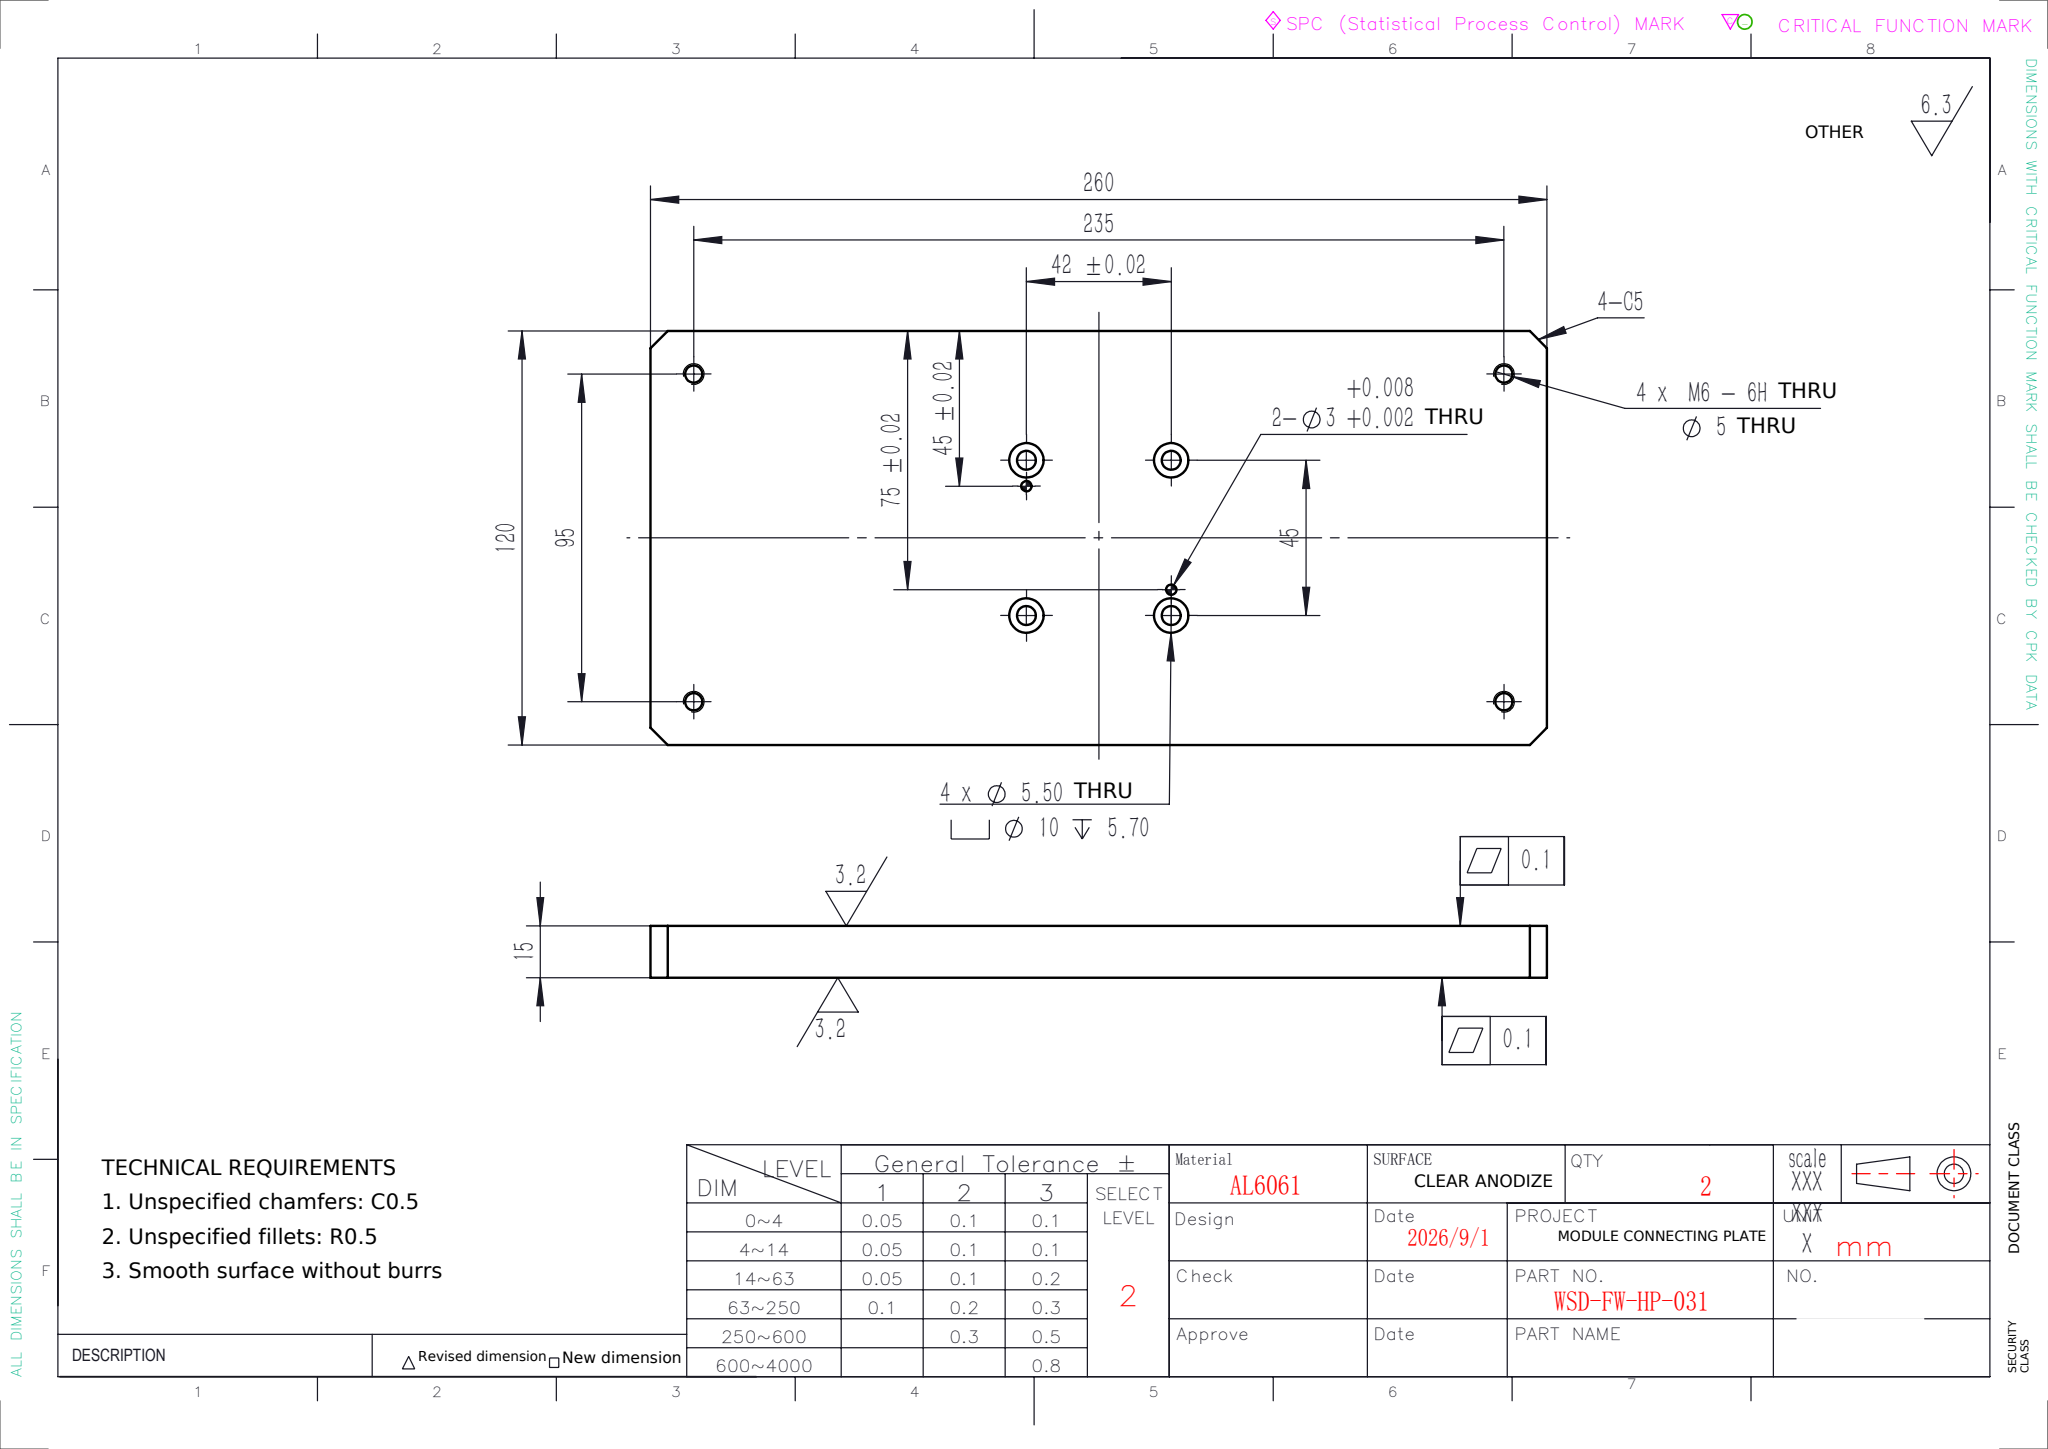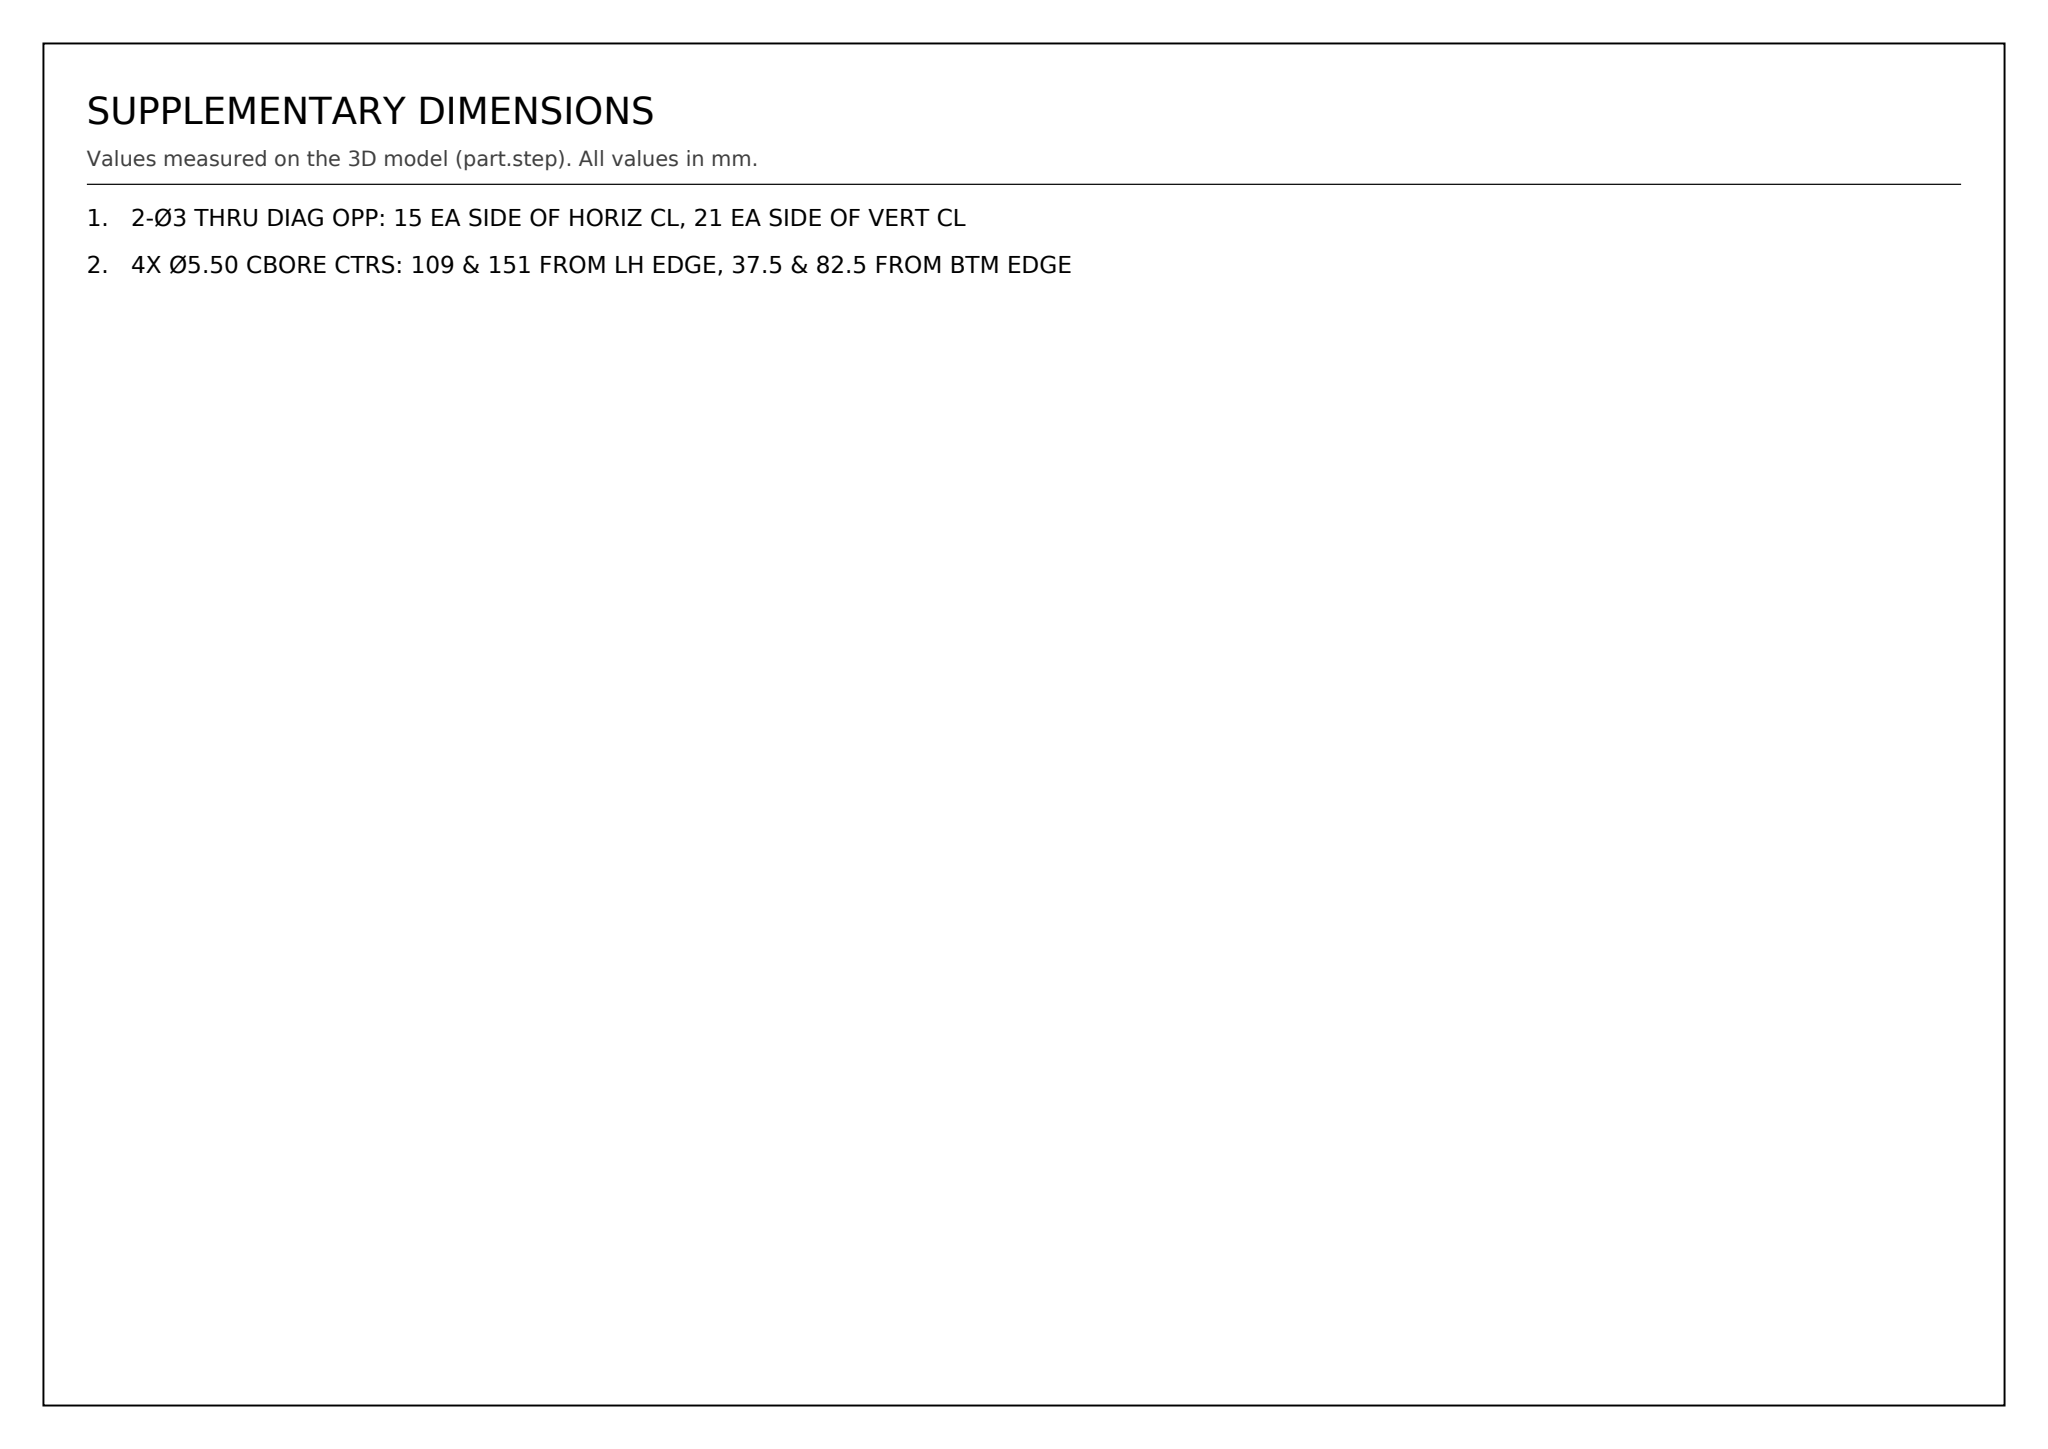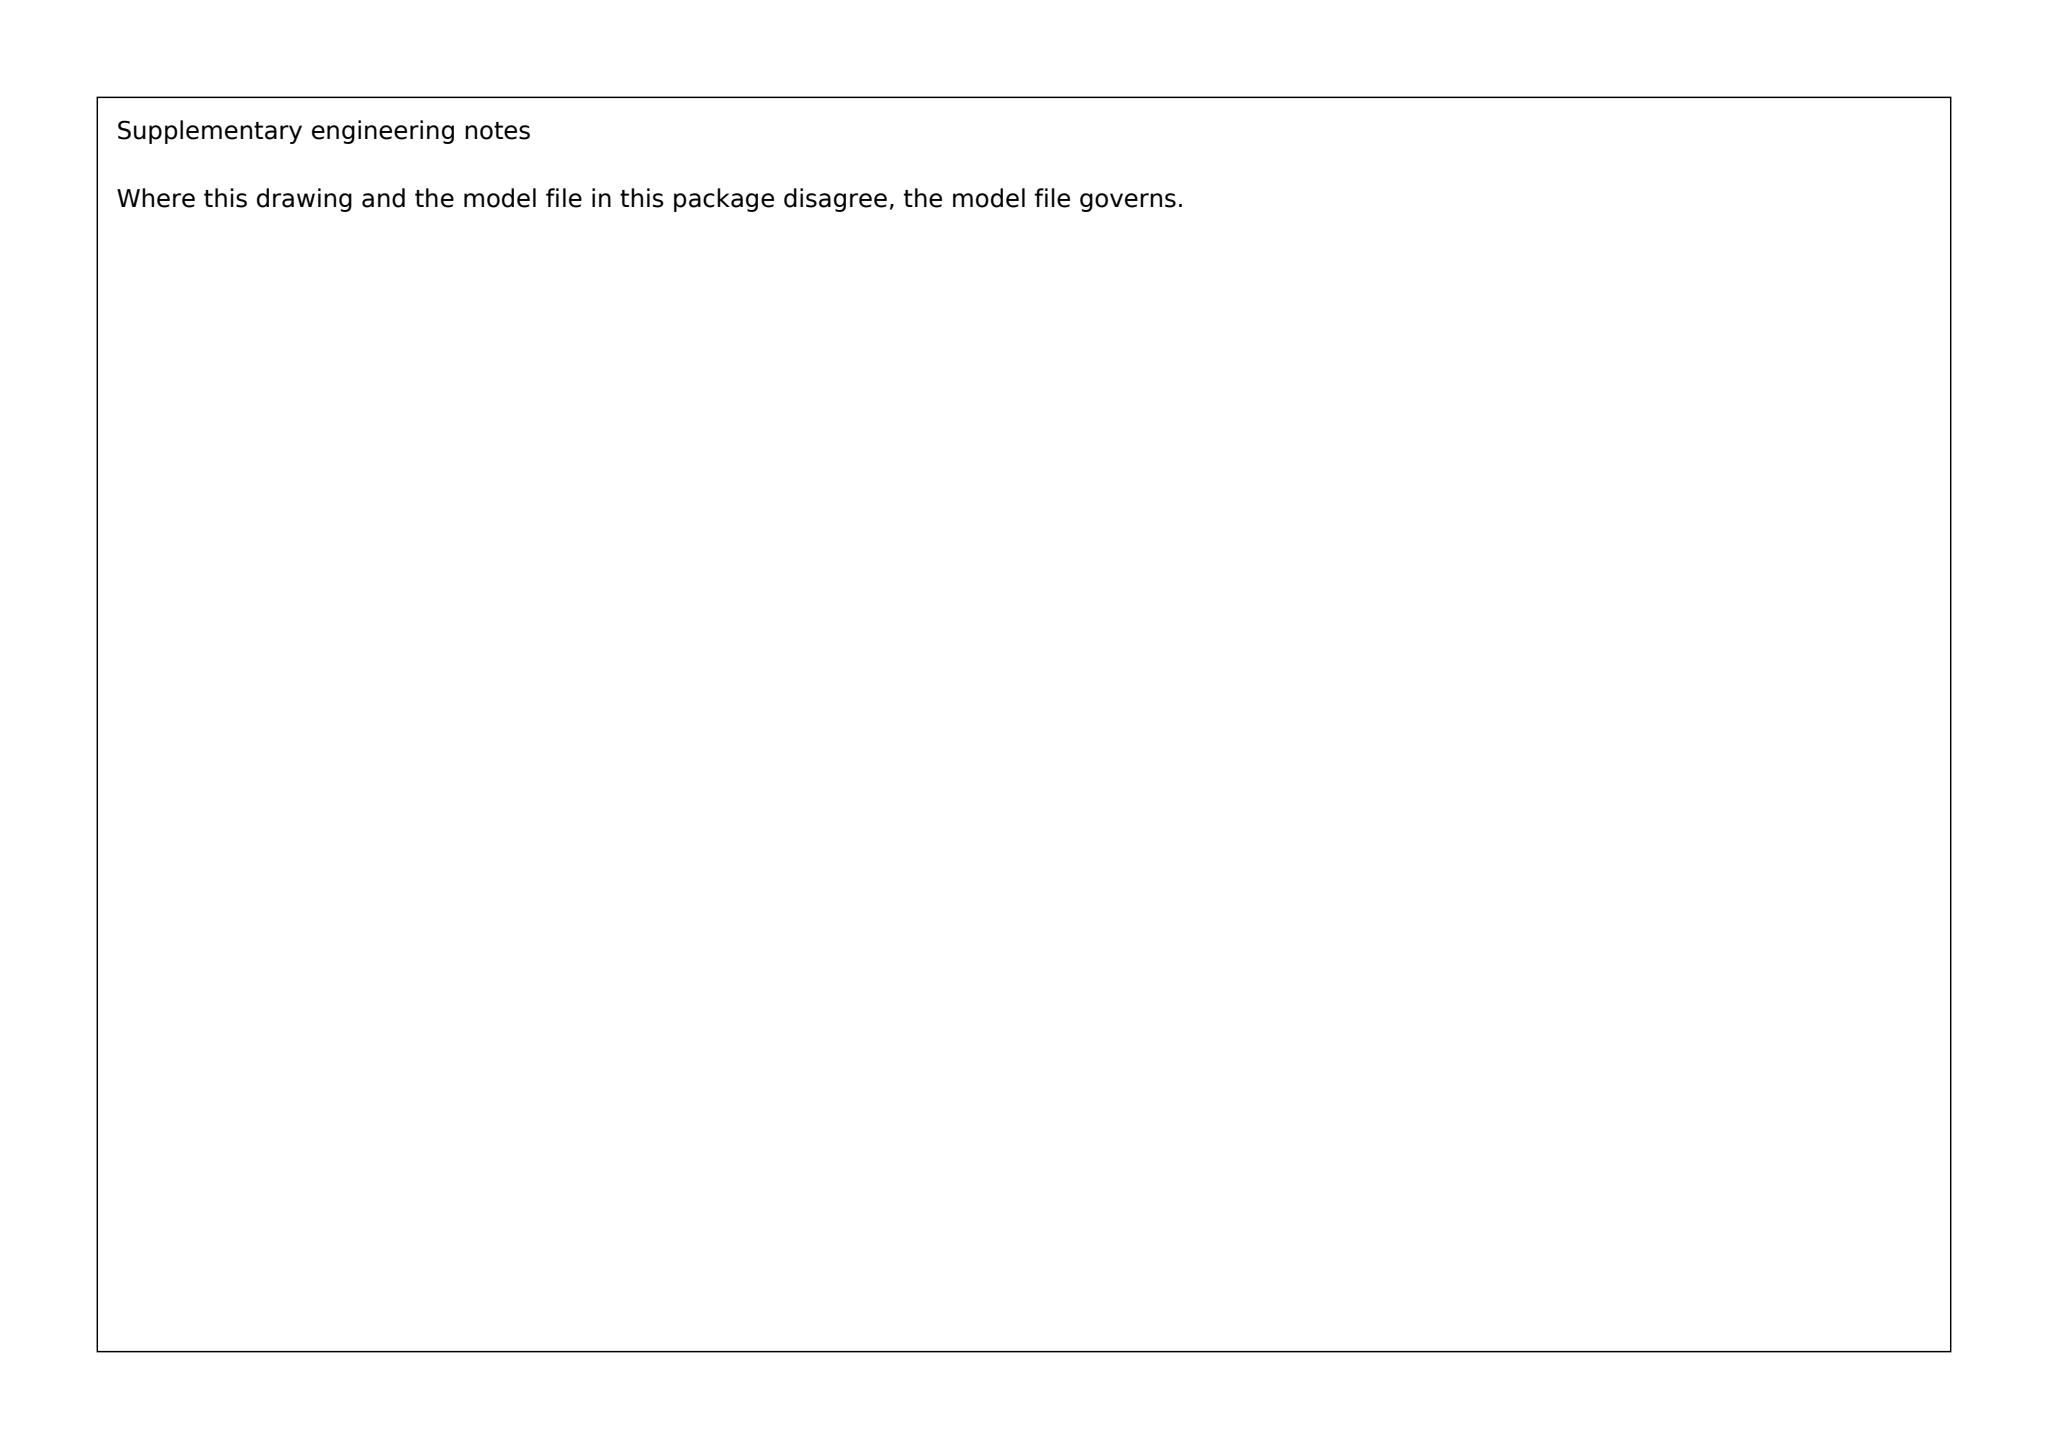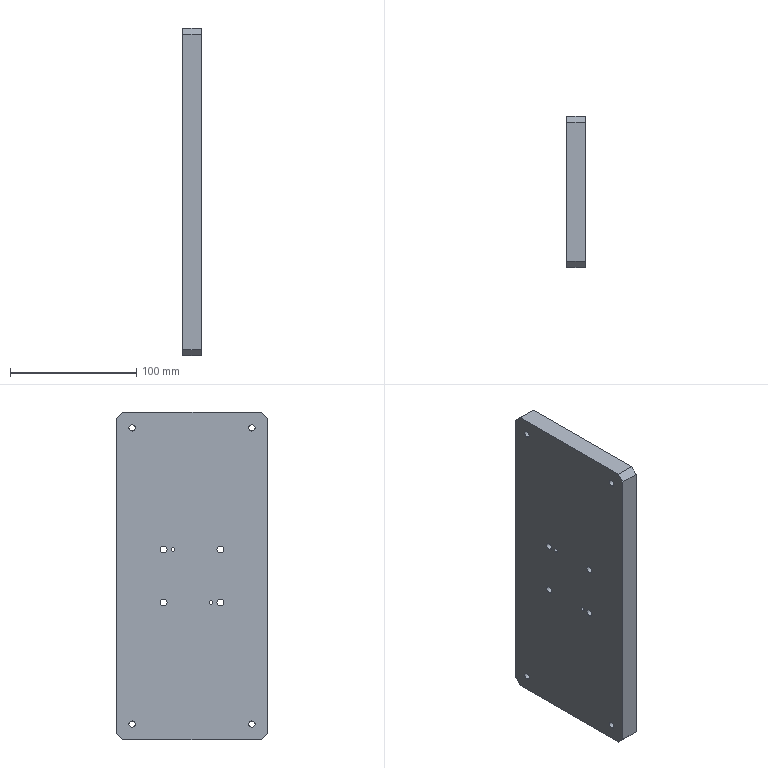Part | SolidWorks | mm | 1 solid | 42 faces | box 15 x 120 x 260 mm | volume 463185 mm3 | cylinder 28 | plane 14 | commonest cylinder face diameters 10 x8 5.5 x8 5 x8 3 x4
Drawing notes:
2-Ø3 THRU DIAG OPP: 15 EA SIDE OF HORIZ CL, 21 EA SIDE OF VERT CL | from the solid: Ø3 x-axis holes at (y,z)=(45,109) & (75,151); plate 120x260, CL y=60/z=130 -> ±15, ±21
4X Ø5.50 CBORE CTRS: 109 & 151 FROM LH EDGE, 37.5 & 82.5 FROM BTM EDGE | from the solid: Ø5.5/Ø10 cbores at z=109 & 151 (42 apart, symm about z=130) and y=37.5 & 82.5
build123d program:
from build123d import *

# Parameters (mm, degrees)
SKETCH1_W                                         = 260
SKETCH1_H                                         = 120
BOSS_EXTRUDE1_DEPTH                               = 15
M6_TAPPED_HOLE1_D                                 = 5
M6_TAPPED_HOLE1_DEPTH                             = 15
M6_TAPPED_HOLE1_TIP                               = 1.502
CHAMFER1_SIZE                                     = 5
HOLE_SIZE_ACCORDING_TO_HEXAGON_SOCKET_D           = 5.5
HOLE_SIZE_ACCORDING_TO_HEXAGON_SOCKET_CBORE_D     = 10
HOLE_SIZE_ACCORDING_TO_HEXAGON_SOCKET_CBORE_DEPTH = 5.7
SKETCH6_R                                         = 1.5
CUT_EXTRUDE1_DEPTH                                = 144.962


with BuildPart() as part:
    # Sketch1 → Boss-Extrude1 (new body)
    with BuildSketch(Plane(origin=(0, 0, 0), x_dir=(0, 0, -1), z_dir=(1, 0, 0))):
        Rectangle(SKETCH1_W, SKETCH1_H)
    extrude(amount=BOSS_EXTRUDE1_DEPTH)

    # M6 Tapped Hole1
    with Locations(Plane(origin=(15, 0, 0), x_dir=(0, 0, -1), z_dir=(1, 0, 0))):
        with Locations((-117.5, 47.5), (117.5, 47.5), (117.5, -47.5), (-117.5, -47.5)):
            Hole(M6_TAPPED_HOLE1_D / 2, depth=M6_TAPPED_HOLE1_DEPTH)
            with Locations((0, 0, -(M6_TAPPED_HOLE1_DEPTH + M6_TAPPED_HOLE1_TIP / 2))):  # 118° drill point
                Cone(0, M6_TAPPED_HOLE1_D / 2, M6_TAPPED_HOLE1_TIP, mode=Mode.SUBTRACT)

    # Chamfer1
    chamfer1_edges = [part.edges().sort_by_distance(p)[0] for p in [
        (7.5, -60, -130),
        (7.5, -60, 130),
        (7.5, 60, 130),
        (7.5, 60, -130),
    ]]
    chamfer(chamfer1_edges, length=CHAMFER1_SIZE)

    # Hole Size _ according to_ Hexagon Socket (through all)
    with Locations(Plane(origin=(15, 0, 0), x_dir=(0, 0, -1), z_dir=(1, 0, 0))):
        with Locations((-21, 22.5), (21, 22.5), (21, -22.5), (-21, -22.5)):
            CounterBoreHole(HOLE_SIZE_ACCORDING_TO_HEXAGON_SOCKET_D / 2, HOLE_SIZE_ACCORDING_TO_HEXAGON_SOCKET_CBORE_D / 2, HOLE_SIZE_ACCORDING_TO_HEXAGON_SOCKET_CBORE_DEPTH)

    # Sketch6 → Cut-Extrude1 (cut, through all)
    with BuildSketch(Plane(origin=(15, 0, 0), x_dir=(0, 0, -1), z_dir=(1, 0, 0))):
        with Locations((-21, 15)):
            Circle(SKETCH6_R)
        with Locations(Location((21, -15, 0), (0, 0, 180))):
            Circle(SKETCH6_R)
    extrude(amount=-CUT_EXTRUDE1_DEPTH, mode=Mode.SUBTRACT)


solid = part.part